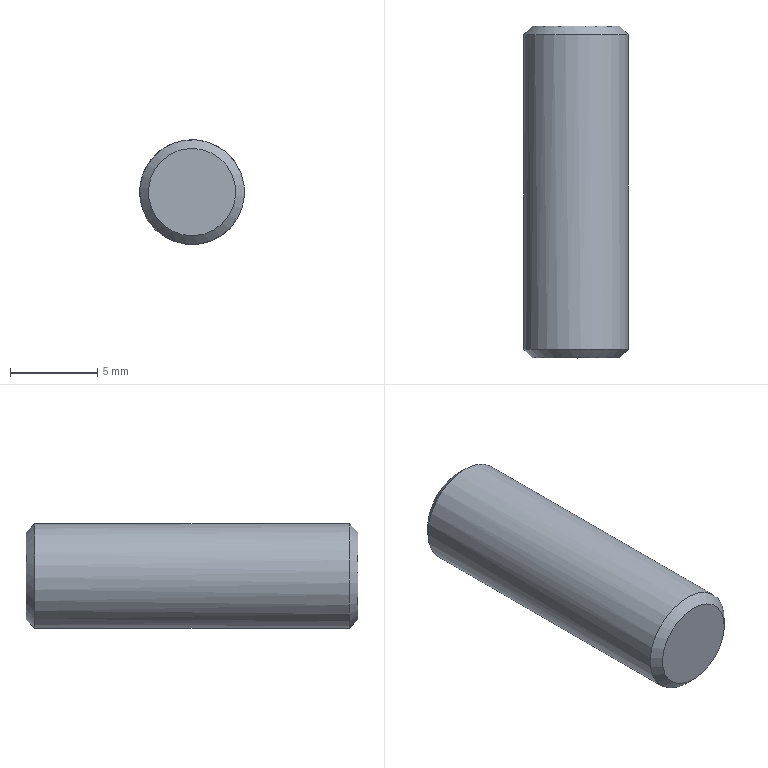Component | NX | PIN | 1 solid | 5 faces | box 6 x 19 x 6 mm | volume 533 mm3 | plane 2 | cone 2 | cylinder 1 | commonest cylinder face diameters 6 x1
STEP:
#1=CARTESIAN_POINT('',(0.,0.,0.));
#2=DIRECTION('',(0.,0.,1.));
#3=DIRECTION('',(1.,0.,0.));
#4=AXIS2_PLACEMENT_3D('',#1,#2,#3);
#5=CARTESIAN_POINT('',(2.491,10.3,79.035));
#6=VERTEX_POINT('',#5);
#7=CARTESIAN_POINT('',(0.0005589,10.3,79.253));
#8=DIRECTION('',(0.,1.,0.));
#9=DIRECTION('',(0.9962,0.,-0.08716));
#10=AXIS2_PLACEMENT_3D('',#7,#8,#9);
#11=CIRCLE('',#10,2.5);
#12=CARTESIAN_POINT('',(0.0005589,10.3,79.253));
#13=DIRECTION('',(0.,1.,0.));
#14=DIRECTION('',(0.9962,0.,-0.08716));
#15=AXIS2_PLACEMENT_3D('',#12,#13,#14);
#16=PLANE('',#15);
#17=CARTESIAN_POINT('',(0.,0.));
#18=DIRECTION('',(1.,-0.));
#19=AXIS2_PLACEMENT_2D('',#17,#18);
#20=CIRCLE('',#19,2.5);
#21=(GEOMETRIC_REPRESENTATION_CONTEXT(2)PARAMETRIC_REPRESENTATION_CONTEXT()REPRESENTATION_CONTEXT('',''));
#22=DEFINITIONAL_REPRESENTATION('',(#20),#21);
#23=PCURVE('',#16,#22);
#24=CARTESIAN_POINT('',(0.0005589,9.8,79.253));
#25=DIRECTION('',(0.,-1.,0.));
#26=DIRECTION('',(-0.9962,0.,0.08716));
#27=AXIS2_PLACEMENT_3D('',#24,#25,#26);
#28=CONICAL_SURFACE('',#27,3.,0.7854);
#29=CARTESIAN_POINT('',(9.425,-0.5));
#30=DIRECTION('',(-1.,0.));
#31=VECTOR('',#30,1.);
#32=LINE('',#29,#31);
#33=(GEOMETRIC_REPRESENTATION_CONTEXT(2)PARAMETRIC_REPRESENTATION_CONTEXT()REPRESENTATION_CONTEXT('',''));
#34=DEFINITIONAL_REPRESENTATION('',(#32),#33);
#35=PCURVE('',#28,#34);
#36=SURFACE_CURVE('',#11,(#23,#35),.PCURVE_S1.);
#37=EDGE_CURVE('',#6,#6,#36,.T.);
#38=ORIENTED_EDGE('',*,*,#37,.T.);
#39=EDGE_LOOP('',(#38));
#40=FACE_BOUND('',#39,.T.);
#41=ADVANCED_FACE('',(#40),#16,.T.);
#42=CARTESIAN_POINT('',(-2.49,-8.7,79.47));
#43=VERTEX_POINT('',#42);
#44=CARTESIAN_POINT('',(0.0005589,-8.7,79.253));
#45=DIRECTION('',(0.,-1.,0.));
#46=DIRECTION('',(-0.9962,0.,0.08716));
#47=AXIS2_PLACEMENT_3D('',#44,#45,#46);
#48=CIRCLE('',#47,2.5);
#49=CARTESIAN_POINT('',(0.0005589,-8.7,79.253));
#50=DIRECTION('',(0.,-1.,0.));
#51=DIRECTION('',(-0.9962,0.,0.08716));
#52=AXIS2_PLACEMENT_3D('',#49,#50,#51);
#53=PLANE('',#52);
#54=CARTESIAN_POINT('',(0.,0.));
#55=DIRECTION('',(1.,0.));
#56=AXIS2_PLACEMENT_2D('',#54,#55);
#57=CIRCLE('',#56,2.5);
#58=(GEOMETRIC_REPRESENTATION_CONTEXT(2)PARAMETRIC_REPRESENTATION_CONTEXT()REPRESENTATION_CONTEXT('',''));
#59=DEFINITIONAL_REPRESENTATION('',(#57),#58);
#60=PCURVE('',#53,#59);
#61=CARTESIAN_POINT('',(0.0005589,-8.2,79.253));
#62=DIRECTION('',(0.,1.,0.));
#63=DIRECTION('',(0.9962,0.,-0.08716));
#64=AXIS2_PLACEMENT_3D('',#61,#62,#63);
#65=CONICAL_SURFACE('',#64,3.,0.7854);
#66=CARTESIAN_POINT('',(9.425,-0.5));
#67=DIRECTION('',(-1.,0.));
#68=VECTOR('',#67,1.);
#69=LINE('',#66,#68);
#70=(GEOMETRIC_REPRESENTATION_CONTEXT(2)PARAMETRIC_REPRESENTATION_CONTEXT()REPRESENTATION_CONTEXT('',''));
#71=DEFINITIONAL_REPRESENTATION('',(#69),#70);
#72=PCURVE('',#65,#71);
#73=SURFACE_CURVE('',#48,(#60,#72),.PCURVE_S1.);
#74=EDGE_CURVE('',#43,#43,#73,.T.);
#75=ORIENTED_EDGE('',*,*,#74,.T.);
#76=EDGE_LOOP('',(#75));
#77=FACE_BOUND('',#76,.T.);
#78=ADVANCED_FACE('',(#77),#53,.T.);
#79=CARTESIAN_POINT('',(-2.988,-8.2,79.514));
#80=VERTEX_POINT('',#79);
#81=CARTESIAN_POINT('',(2.989,-8.2,78.991));
#82=VERTEX_POINT('',#81);
#83=CARTESIAN_POINT('',(0.0005589,-8.2,79.253));
#84=DIRECTION('',(0.,1.,0.));
#85=DIRECTION('',(-0.9962,0.,0.08716));
#86=AXIS2_PLACEMENT_3D('',#83,#84,#85);
#87=CIRCLE('',#86,3.);
#88=CARTESIAN_POINT('',(0.0005589,-8.7,79.253));
#89=DIRECTION('',(0.,1.,0.));
#90=DIRECTION('',(0.9962,0.,-0.08716));
#91=AXIS2_PLACEMENT_3D('',#88,#89,#90);
#92=CYLINDRICAL_SURFACE('',#91,3.);
#93=CARTESIAN_POINT('',(3.142,0.5));
#94=DIRECTION('',(1.,0.));
#95=VECTOR('',#94,1.);
#96=LINE('',#93,#95);
#97=(GEOMETRIC_REPRESENTATION_CONTEXT(2)PARAMETRIC_REPRESENTATION_CONTEXT()REPRESENTATION_CONTEXT('',''));
#98=DEFINITIONAL_REPRESENTATION('',(#96),#97);
#99=PCURVE('',#92,#98);
#100=CARTESIAN_POINT('',(3.142,0.));
#101=DIRECTION('',(1.,-0.));
#102=VECTOR('',#101,1.);
#103=LINE('',#100,#102);
#104=(GEOMETRIC_REPRESENTATION_CONTEXT(2)PARAMETRIC_REPRESENTATION_CONTEXT()REPRESENTATION_CONTEXT('',''));
#105=DEFINITIONAL_REPRESENTATION('',(#103),#104);
#106=PCURVE('',#65,#105);
#107=SURFACE_CURVE('',#87,(#99,#106),.PCURVE_S1.);
#108=EDGE_CURVE('',#80,#82,#107,.T.);
#109=ORIENTED_EDGE('',*,*,#108,.T.);
#110=CARTESIAN_POINT('',(2.989,9.8,78.991));
#111=VERTEX_POINT('',#110);
#112=CARTESIAN_POINT('',(2.989,-8.2,78.991));
#113=CARTESIAN_POINT('',(2.989,9.8,78.991));
#114=B_SPLINE_CURVE_WITH_KNOTS('',1,(#112,#113),.UNSPECIFIED.,.F.,.F.,(2,2),(0.5,18.5),.PIECEWISE_BEZIER_KNOTS.);
#115=CARTESIAN_POINT('',(6.283,0.));
#116=DIRECTION('',(0.,1.));
#117=VECTOR('',#116,1.);
#118=LINE('',#115,#117);
#119=(GEOMETRIC_REPRESENTATION_CONTEXT(2)PARAMETRIC_REPRESENTATION_CONTEXT()REPRESENTATION_CONTEXT('',''));
#120=DEFINITIONAL_REPRESENTATION('',(#118),#119);
#121=PCURVE('',#92,#120);
#122=CARTESIAN_POINT('',(0.,0.));
#123=DIRECTION('',(0.,1.));
#124=VECTOR('',#123,1.);
#125=LINE('',#122,#124);
#126=(GEOMETRIC_REPRESENTATION_CONTEXT(2)PARAMETRIC_REPRESENTATION_CONTEXT()REPRESENTATION_CONTEXT('',''));
#127=DEFINITIONAL_REPRESENTATION('',(#125),#126);
#128=PCURVE('',#92,#127);
#129=SEAM_CURVE('',#114,(#121,#128),.PCURVE_S1.);
#130=EDGE_CURVE('',#82,#111,#129,.T.);
#131=ORIENTED_EDGE('',*,*,#130,.T.);
#132=CARTESIAN_POINT('',(0.0005589,9.8,79.253));
#133=DIRECTION('',(0.,-1.,0.));
#134=DIRECTION('',(0.9962,0.,-0.08716));
#135=AXIS2_PLACEMENT_3D('',#132,#133,#134);
#136=CIRCLE('',#135,3.);
#137=CARTESIAN_POINT('',(6.283,18.5));
#138=DIRECTION('',(-1.,0.));
#139=VECTOR('',#138,1.);
#140=LINE('',#137,#139);
#141=(GEOMETRIC_REPRESENTATION_CONTEXT(2)PARAMETRIC_REPRESENTATION_CONTEXT()REPRESENTATION_CONTEXT('',''));
#142=DEFINITIONAL_REPRESENTATION('',(#140),#141);
#143=PCURVE('',#92,#142);
#144=CARTESIAN_POINT('',(3.142,-0.));
#145=DIRECTION('',(1.,0.));
#146=VECTOR('',#145,1.);
#147=LINE('',#144,#146);
#148=(GEOMETRIC_REPRESENTATION_CONTEXT(2)PARAMETRIC_REPRESENTATION_CONTEXT()REPRESENTATION_CONTEXT('',''));
#149=DEFINITIONAL_REPRESENTATION('',(#147),#148);
#150=PCURVE('',#28,#149);
#151=SURFACE_CURVE('',#136,(#143,#150),.PCURVE_S1.);
#152=EDGE_CURVE('',#111,#111,#151,.T.);
#153=ORIENTED_EDGE('',*,*,#152,.T.);
#154=ORIENTED_EDGE('',*,*,#130,.F.);
#155=CARTESIAN_POINT('',(0.0005589,-8.2,79.253));
#156=DIRECTION('',(0.,1.,0.));
#157=DIRECTION('',(-0.9962,0.,0.08716));
#158=AXIS2_PLACEMENT_3D('',#155,#156,#157);
#159=CIRCLE('',#158,3.);
#160=CARTESIAN_POINT('',(-3.142,0.5));
#161=DIRECTION('',(1.,0.));
#162=VECTOR('',#161,1.);
#163=LINE('',#160,#162);
#164=(GEOMETRIC_REPRESENTATION_CONTEXT(2)PARAMETRIC_REPRESENTATION_CONTEXT()REPRESENTATION_CONTEXT('',''));
#165=DEFINITIONAL_REPRESENTATION('',(#163),#164);
#166=PCURVE('',#92,#165);
#167=CARTESIAN_POINT('',(3.142,-0.));
#168=DIRECTION('',(1.,0.));
#169=VECTOR('',#168,1.);
#170=LINE('',#167,#169);
#171=(GEOMETRIC_REPRESENTATION_CONTEXT(2)PARAMETRIC_REPRESENTATION_CONTEXT()REPRESENTATION_CONTEXT('',''));
#172=DEFINITIONAL_REPRESENTATION('',(#170),#171);
#173=PCURVE('',#65,#172);
#174=SURFACE_CURVE('',#159,(#166,#173),.PCURVE_S1.);
#175=EDGE_CURVE('',#82,#80,#174,.T.);
#176=ORIENTED_EDGE('',*,*,#175,.T.);
#177=EDGE_LOOP('',(#109,#131,#153,#154,#176));
#178=FACE_BOUND('',#177,.T.);
#179=ADVANCED_FACE('',(#178),#92,.T.);
#180=ORIENTED_EDGE('',*,*,#74,.F.);
#181=CARTESIAN_POINT('',(-2.49,-8.7,79.47));
#182=CARTESIAN_POINT('',(-2.988,-8.2,79.514));
#183=B_SPLINE_CURVE_WITH_KNOTS('',1,(#181,#182),.UNSPECIFIED.,.F.,.F.,(2,2),(-0.7071,0.),.PIECEWISE_BEZIER_KNOTS.);
#184=CARTESIAN_POINT('',(9.425,0.));
#185=DIRECTION('',(0.,1.));
#186=VECTOR('',#185,1.);
#187=LINE('',#184,#186);
#188=(GEOMETRIC_REPRESENTATION_CONTEXT(2)PARAMETRIC_REPRESENTATION_CONTEXT()REPRESENTATION_CONTEXT('',''));
#189=DEFINITIONAL_REPRESENTATION('',(#187),#188);
#190=PCURVE('',#65,#189);
#191=CARTESIAN_POINT('',(3.142,0.));
#192=DIRECTION('',(0.,1.));
#193=VECTOR('',#192,1.);
#194=LINE('',#191,#193);
#195=(GEOMETRIC_REPRESENTATION_CONTEXT(2)PARAMETRIC_REPRESENTATION_CONTEXT()REPRESENTATION_CONTEXT('',''));
#196=DEFINITIONAL_REPRESENTATION('',(#194),#195);
#197=PCURVE('',#65,#196);
#198=SEAM_CURVE('',#183,(#190,#197),.PCURVE_S1.);
#199=EDGE_CURVE('',#43,#80,#198,.T.);
#200=ORIENTED_EDGE('',*,*,#199,.T.);
#201=ORIENTED_EDGE('',*,*,#175,.F.);
#202=ORIENTED_EDGE('',*,*,#108,.F.);
#203=ORIENTED_EDGE('',*,*,#199,.F.);
#204=EDGE_LOOP('',(#180,#200,#201,#202,#203));
#205=FACE_BOUND('',#204,.T.);
#206=ADVANCED_FACE('',(#205),#65,.T.);
#207=ORIENTED_EDGE('',*,*,#37,.F.);
#208=CARTESIAN_POINT('',(2.491,10.3,79.035));
#209=CARTESIAN_POINT('',(2.989,9.8,78.991));
#210=B_SPLINE_CURVE_WITH_KNOTS('',1,(#208,#209),.UNSPECIFIED.,.F.,.F.,(2,2),(-0.7071,-0.),.PIECEWISE_BEZIER_KNOTS.);
#211=CARTESIAN_POINT('',(9.425,0.));
#212=DIRECTION('',(0.,1.));
#213=VECTOR('',#212,1.);
#214=LINE('',#211,#213);
#215=(GEOMETRIC_REPRESENTATION_CONTEXT(2)PARAMETRIC_REPRESENTATION_CONTEXT()REPRESENTATION_CONTEXT('',''));
#216=DEFINITIONAL_REPRESENTATION('',(#214),#215);
#217=PCURVE('',#28,#216);
#218=CARTESIAN_POINT('',(3.142,0.));
#219=DIRECTION('',(0.,1.));
#220=VECTOR('',#219,1.);
#221=LINE('',#218,#220);
#222=(GEOMETRIC_REPRESENTATION_CONTEXT(2)PARAMETRIC_REPRESENTATION_CONTEXT()REPRESENTATION_CONTEXT('',''));
#223=DEFINITIONAL_REPRESENTATION('',(#221),#222);
#224=PCURVE('',#28,#223);
#225=SEAM_CURVE('',#210,(#217,#224),.PCURVE_S1.);
#226=EDGE_CURVE('',#6,#111,#225,.T.);
#227=ORIENTED_EDGE('',*,*,#226,.T.);
#228=ORIENTED_EDGE('',*,*,#152,.F.);
#229=ORIENTED_EDGE('',*,*,#226,.F.);
#230=EDGE_LOOP('',(#207,#227,#228,#229));
#231=FACE_BOUND('',#230,.T.);
#232=ADVANCED_FACE('',(#231),#28,.T.);
#233=CLOSED_SHELL('',(#41,#78,#179,#206,#232));
#234=MANIFOLD_SOLID_BREP('',#233);
#235=(LENGTH_UNIT()NAMED_UNIT(*)SI_UNIT(.MILLI.,.METRE.));
#236=UNCERTAINTY_MEASURE_WITH_UNIT(LENGTH_MEASURE(0.00001),#235,'','');
#237=(NAMED_UNIT(*)PLANE_ANGLE_UNIT()SI_UNIT($,.RADIAN.));
#238=(NAMED_UNIT(*)SI_UNIT($,.STERADIAN.)SOLID_ANGLE_UNIT());
#239=(GEOMETRIC_REPRESENTATION_CONTEXT(3)GLOBAL_UNCERTAINTY_ASSIGNED_CONTEXT((#236))GLOBAL_UNIT_ASSIGNED_CONTEXT((#235,#237,#238))REPRESENTATION_CONTEXT('',''));
#240=ADVANCED_BREP_SHAPE_REPRESENTATION('',(#4,#234),#239);